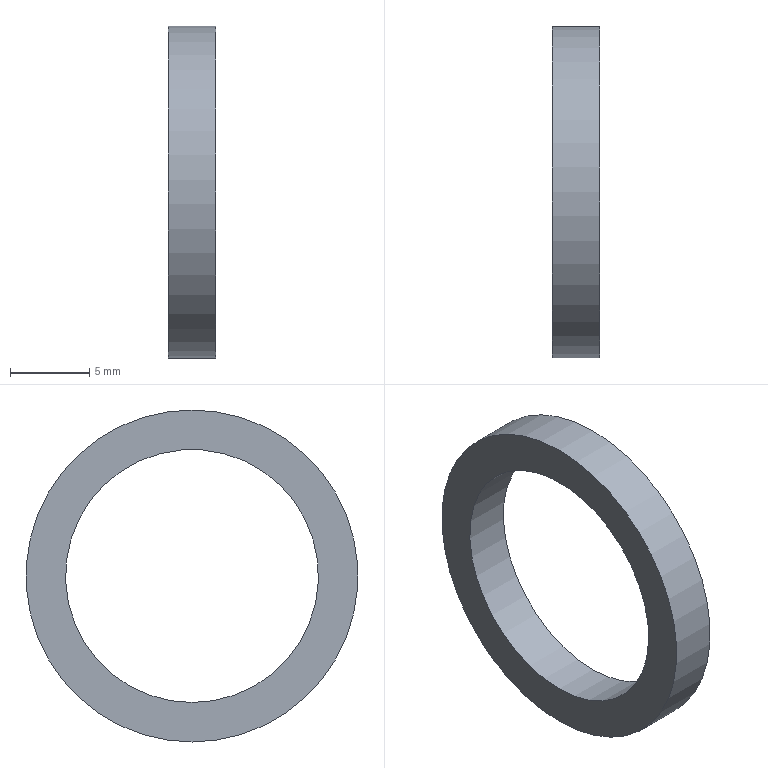Component | NX | END_CAP_4_WASHER | 1 solid | 4 faces | volume 436 mm3 | cylinder 2 | plane 2 | commonest cylinder face diameters 21 x1 16 x1